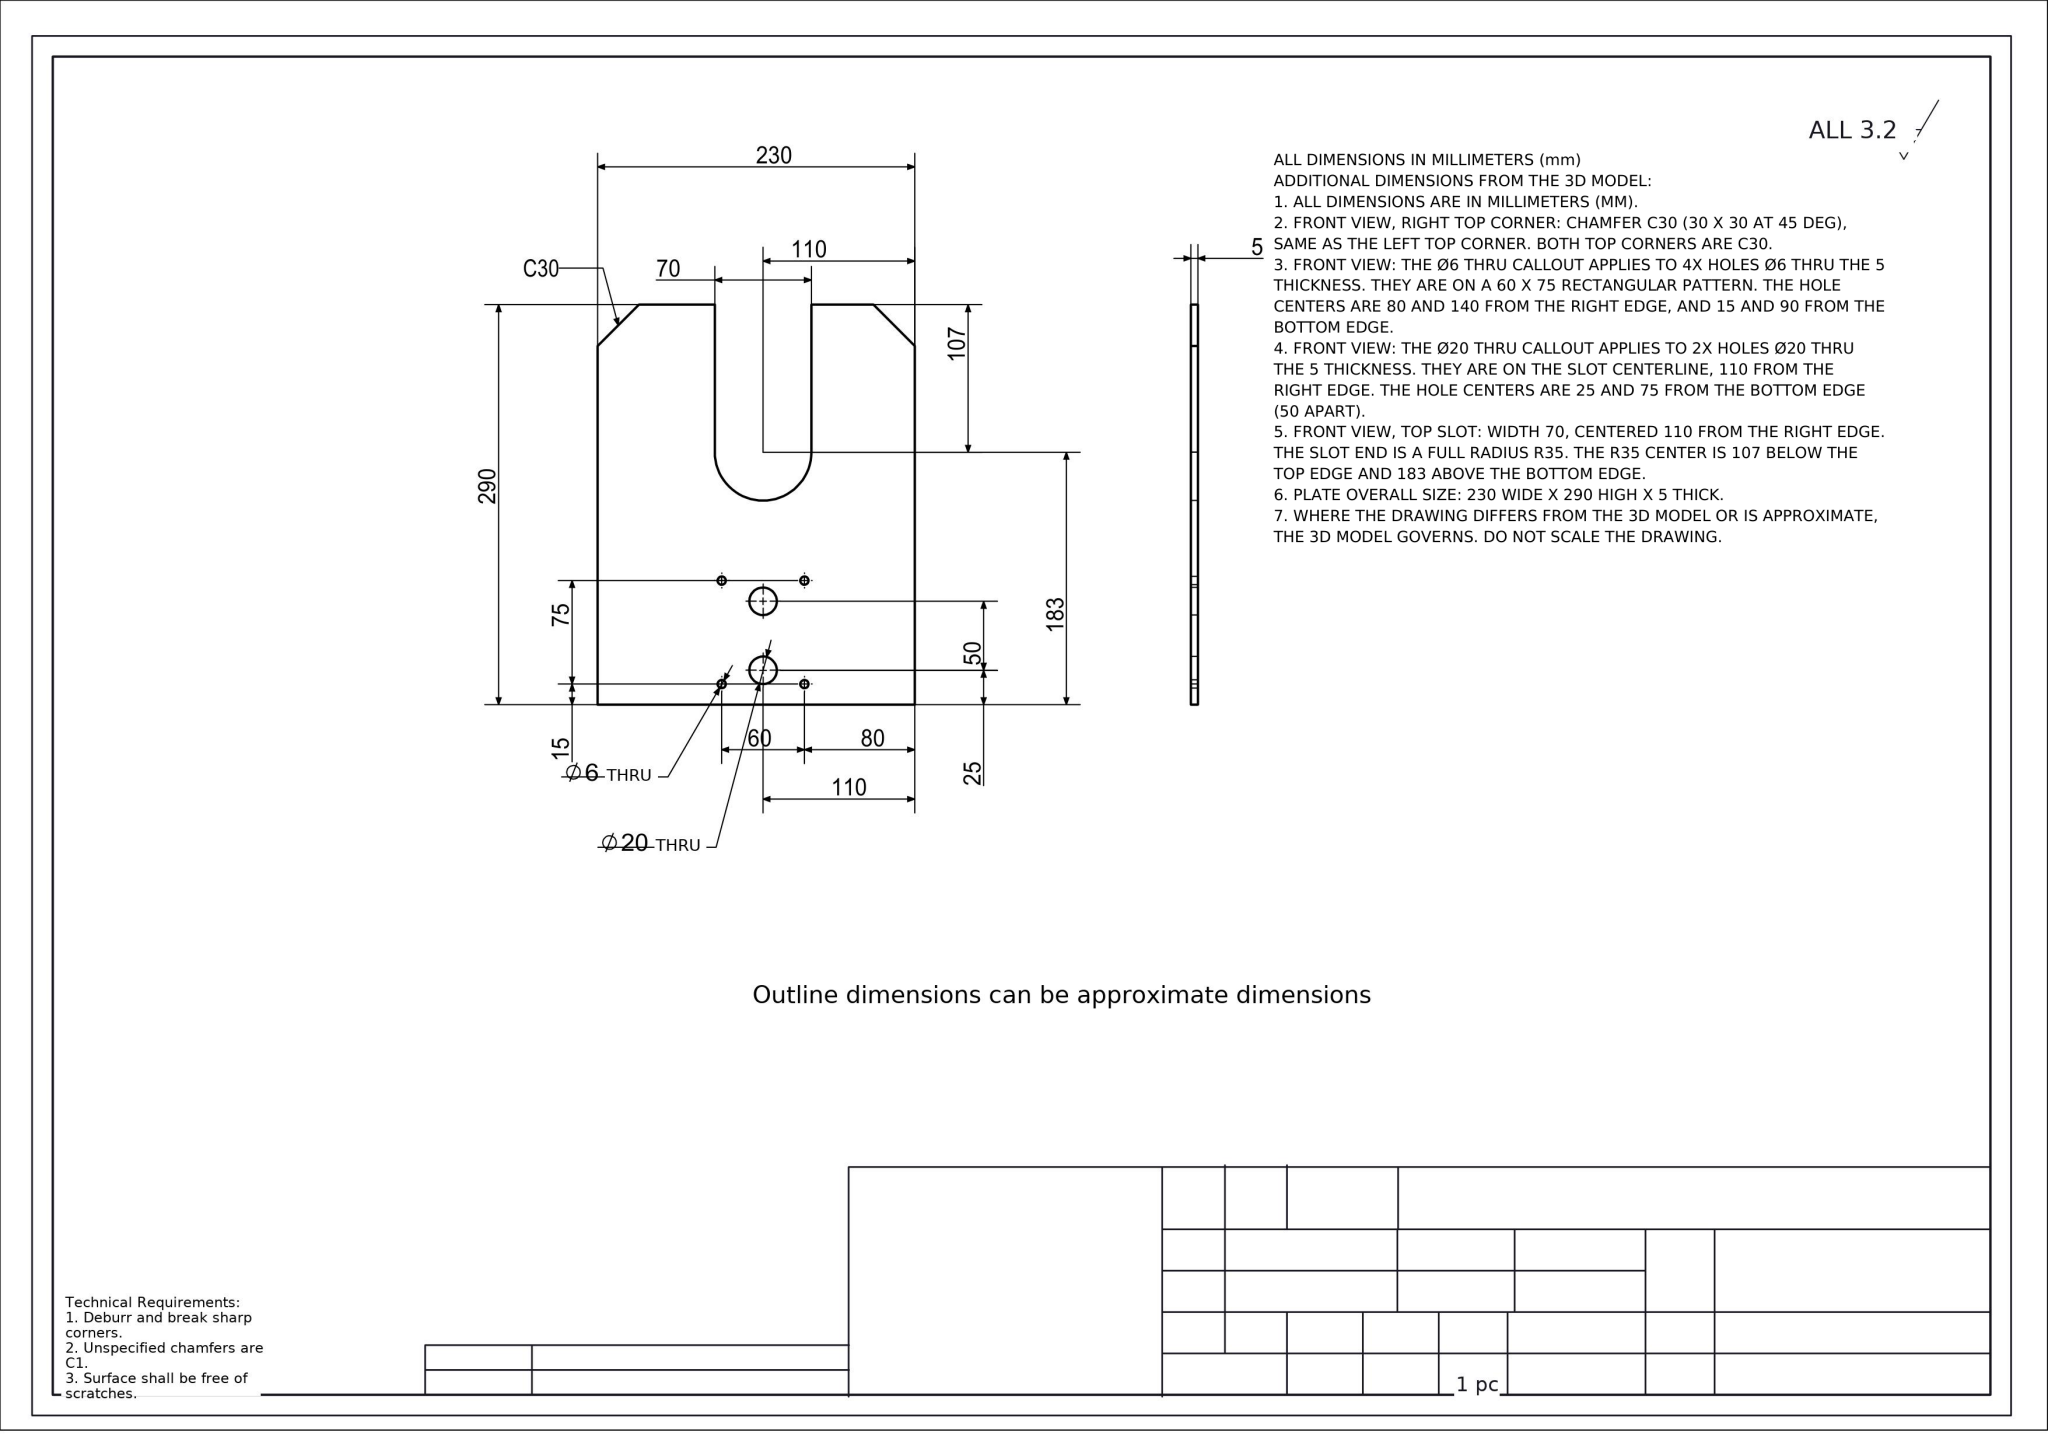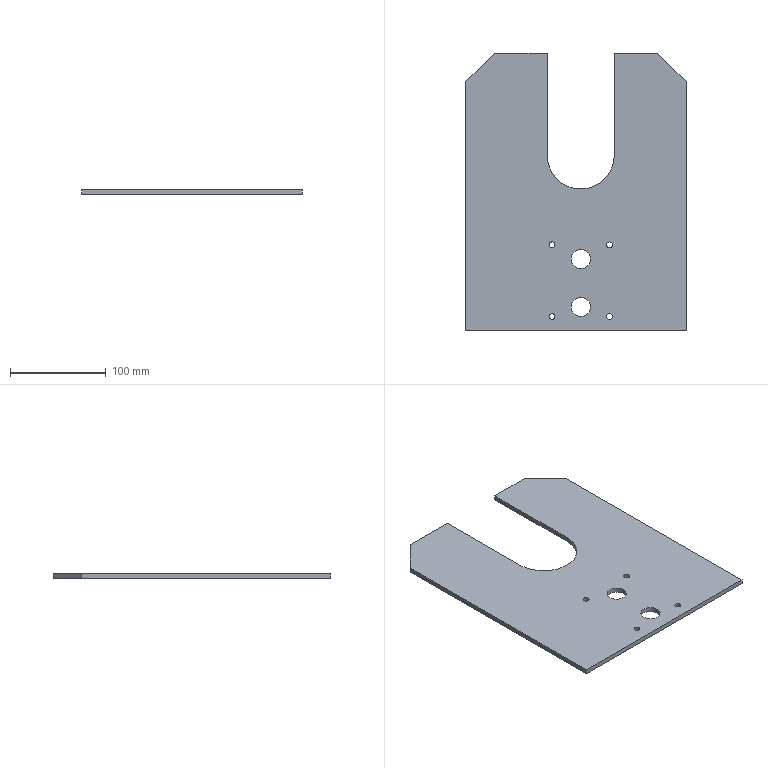Part | NX | mm | U-Notched Multi-Bore Base Plate 230mm | 1 solid | 24 faces | box 230 x 290 x 5 mm | volume 278222 mm3 | cylinder 13 | plane 11 | commonest cylinder face diameters 6 x8 20 x4 70 x1
STEP:
#1=COLOUR_RGB('',0.7922,0.8196,0.9333);
#2=FILL_AREA_STYLE_COLOUR('',#1);
#3=FILL_AREA_STYLE('',(#2));
#4=SURFACE_STYLE_FILL_AREA(#3);
#5=SURFACE_SIDE_STYLE('',(#4));
#6=SURFACE_STYLE_USAGE(.BOTH.,#5);
#7=PRESENTATION_STYLE_ASSIGNMENT((#6));
#8=CARTESIAN_POINT('',(-7.627,5.308,0.));
#9=VERTEX_POINT('',#8);
#10=CARTESIAN_POINT('',(-1.627,5.308,0.));
#11=VERTEX_POINT('',#10);
#12=CARTESIAN_POINT('',(-4.627,5.308,0.));
#13=DIRECTION('',(0.,0.,1.));
#14=DIRECTION('',(1.,0.,0.));
#15=AXIS2_PLACEMENT_3D('',#12,#13,#14);
#16=CIRCLE('',#15,3.);
#17=EDGE_CURVE('',#9,#11,#16,.T.);
#18=ORIENTED_EDGE('',*,*,#17,.F.);
#19=CARTESIAN_POINT('',(-7.627,5.308,5.));
#20=VERTEX_POINT('',#19);
#21=CARTESIAN_POINT('',(-7.627,5.308,0.));
#22=DIRECTION('',(0.,0.,1.));
#23=VECTOR('',#22,1000.);
#24=LINE('',#21,#23);
#25=EDGE_CURVE('',#9,#20,#24,.T.);
#26=ORIENTED_EDGE('',*,*,#25,.T.);
#27=CARTESIAN_POINT('',(-1.627,5.308,5.));
#28=VERTEX_POINT('',#27);
#29=CARTESIAN_POINT('',(-4.627,5.308,5.));
#30=DIRECTION('',(0.,0.,1.));
#31=DIRECTION('',(1.,0.,0.));
#32=AXIS2_PLACEMENT_3D('',#29,#30,#31);
#33=CIRCLE('',#32,3.);
#34=EDGE_CURVE('',#20,#28,#33,.T.);
#35=ORIENTED_EDGE('',*,*,#34,.T.);
#36=CARTESIAN_POINT('',(-1.627,5.308,0.));
#37=DIRECTION('',(0.,0.,1.));
#38=VECTOR('',#37,1000.);
#39=LINE('',#36,#38);
#40=EDGE_CURVE('',#11,#28,#39,.T.);
#41=ORIENTED_EDGE('',*,*,#40,.F.);
#42=EDGE_LOOP('',(#18,#26,#35,#41));
#43=FACE_OUTER_BOUND('',#42,.T.);
#44=CARTESIAN_POINT('',(-4.627,5.308,0.));
#45=DIRECTION('',(0.,0.,1.));
#46=DIRECTION('',(1.,0.,0.));
#47=AXIS2_PLACEMENT_3D('',#44,#45,#46);
#48=CYLINDRICAL_SURFACE('',#47,3.);
#49=ADVANCED_FACE('',(#43),#48,.F.);
#50=CARTESIAN_POINT('',(-7.627,80.308,0.));
#51=VERTEX_POINT('',#50);
#52=CARTESIAN_POINT('',(-1.627,80.308,0.));
#53=VERTEX_POINT('',#52);
#54=CARTESIAN_POINT('',(-4.627,80.308,0.));
#55=DIRECTION('',(0.,0.,1.));
#56=DIRECTION('',(1.,0.,0.));
#57=AXIS2_PLACEMENT_3D('',#54,#55,#56);
#58=CIRCLE('',#57,3.);
#59=EDGE_CURVE('',#51,#53,#58,.T.);
#60=ORIENTED_EDGE('',*,*,#59,.F.);
#61=CARTESIAN_POINT('',(-7.627,80.308,5.));
#62=VERTEX_POINT('',#61);
#63=CARTESIAN_POINT('',(-7.627,80.308,0.));
#64=DIRECTION('',(0.,0.,1.));
#65=VECTOR('',#64,1000.);
#66=LINE('',#63,#65);
#67=EDGE_CURVE('',#51,#62,#66,.T.);
#68=ORIENTED_EDGE('',*,*,#67,.T.);
#69=CARTESIAN_POINT('',(-1.627,80.308,5.));
#70=VERTEX_POINT('',#69);
#71=CARTESIAN_POINT('',(-4.627,80.308,5.));
#72=DIRECTION('',(0.,0.,1.));
#73=DIRECTION('',(1.,0.,0.));
#74=AXIS2_PLACEMENT_3D('',#71,#72,#73);
#75=CIRCLE('',#74,3.);
#76=EDGE_CURVE('',#62,#70,#75,.T.);
#77=ORIENTED_EDGE('',*,*,#76,.T.);
#78=CARTESIAN_POINT('',(-1.627,80.308,0.));
#79=DIRECTION('',(0.,0.,1.));
#80=VECTOR('',#79,1000.);
#81=LINE('',#78,#80);
#82=EDGE_CURVE('',#53,#70,#81,.T.);
#83=ORIENTED_EDGE('',*,*,#82,.F.);
#84=EDGE_LOOP('',(#60,#68,#77,#83));
#85=FACE_OUTER_BOUND('',#84,.T.);
#86=CARTESIAN_POINT('',(-4.627,80.308,0.));
#87=DIRECTION('',(0.,0.,1.));
#88=DIRECTION('',(1.,0.,0.));
#89=AXIS2_PLACEMENT_3D('',#86,#87,#88);
#90=CYLINDRICAL_SURFACE('',#89,3.);
#91=ADVANCED_FACE('',(#85),#90,.F.);
#92=CARTESIAN_POINT('',(52.373,5.308,0.));
#93=VERTEX_POINT('',#92);
#94=CARTESIAN_POINT('',(58.373,5.308,0.));
#95=VERTEX_POINT('',#94);
#96=CARTESIAN_POINT('',(55.373,5.308,0.));
#97=DIRECTION('',(0.,0.,1.));
#98=DIRECTION('',(1.,0.,0.));
#99=AXIS2_PLACEMENT_3D('',#96,#97,#98);
#100=CIRCLE('',#99,3.);
#101=EDGE_CURVE('',#93,#95,#100,.T.);
#102=ORIENTED_EDGE('',*,*,#101,.F.);
#103=CARTESIAN_POINT('',(52.373,5.308,5.));
#104=VERTEX_POINT('',#103);
#105=CARTESIAN_POINT('',(52.373,5.308,0.));
#106=DIRECTION('',(0.,0.,1.));
#107=VECTOR('',#106,1000.);
#108=LINE('',#105,#107);
#109=EDGE_CURVE('',#93,#104,#108,.T.);
#110=ORIENTED_EDGE('',*,*,#109,.T.);
#111=CARTESIAN_POINT('',(58.373,5.308,5.));
#112=VERTEX_POINT('',#111);
#113=CARTESIAN_POINT('',(55.373,5.308,5.));
#114=DIRECTION('',(0.,0.,1.));
#115=DIRECTION('',(1.,0.,0.));
#116=AXIS2_PLACEMENT_3D('',#113,#114,#115);
#117=CIRCLE('',#116,3.);
#118=EDGE_CURVE('',#104,#112,#117,.T.);
#119=ORIENTED_EDGE('',*,*,#118,.T.);
#120=CARTESIAN_POINT('',(58.373,5.308,0.));
#121=DIRECTION('',(0.,0.,1.));
#122=VECTOR('',#121,1000.);
#123=LINE('',#120,#122);
#124=EDGE_CURVE('',#95,#112,#123,.T.);
#125=ORIENTED_EDGE('',*,*,#124,.F.);
#126=EDGE_LOOP('',(#102,#110,#119,#125));
#127=FACE_OUTER_BOUND('',#126,.T.);
#128=CARTESIAN_POINT('',(55.373,5.308,0.));
#129=DIRECTION('',(0.,0.,1.));
#130=DIRECTION('',(1.,0.,0.));
#131=AXIS2_PLACEMENT_3D('',#128,#129,#130);
#132=CYLINDRICAL_SURFACE('',#131,3.);
#133=ADVANCED_FACE('',(#127),#132,.F.);
#134=CARTESIAN_POINT('',(52.373,80.308,0.));
#135=VERTEX_POINT('',#134);
#136=CARTESIAN_POINT('',(58.373,80.308,0.));
#137=VERTEX_POINT('',#136);
#138=CARTESIAN_POINT('',(55.373,80.308,0.));
#139=DIRECTION('',(0.,0.,1.));
#140=DIRECTION('',(1.,0.,0.));
#141=AXIS2_PLACEMENT_3D('',#138,#139,#140);
#142=CIRCLE('',#141,3.);
#143=EDGE_CURVE('',#135,#137,#142,.T.);
#144=ORIENTED_EDGE('',*,*,#143,.F.);
#145=CARTESIAN_POINT('',(52.373,80.308,5.));
#146=VERTEX_POINT('',#145);
#147=CARTESIAN_POINT('',(52.373,80.308,0.));
#148=DIRECTION('',(0.,0.,1.));
#149=VECTOR('',#148,1000.);
#150=LINE('',#147,#149);
#151=EDGE_CURVE('',#135,#146,#150,.T.);
#152=ORIENTED_EDGE('',*,*,#151,.T.);
#153=CARTESIAN_POINT('',(58.373,80.308,5.));
#154=VERTEX_POINT('',#153);
#155=CARTESIAN_POINT('',(55.373,80.308,5.));
#156=DIRECTION('',(0.,0.,1.));
#157=DIRECTION('',(1.,0.,0.));
#158=AXIS2_PLACEMENT_3D('',#155,#156,#157);
#159=CIRCLE('',#158,3.);
#160=EDGE_CURVE('',#146,#154,#159,.T.);
#161=ORIENTED_EDGE('',*,*,#160,.T.);
#162=CARTESIAN_POINT('',(58.373,80.308,0.));
#163=DIRECTION('',(0.,0.,1.));
#164=VECTOR('',#163,1000.);
#165=LINE('',#162,#164);
#166=EDGE_CURVE('',#137,#154,#165,.T.);
#167=ORIENTED_EDGE('',*,*,#166,.F.);
#168=EDGE_LOOP('',(#144,#152,#161,#167));
#169=FACE_OUTER_BOUND('',#168,.T.);
#170=CARTESIAN_POINT('',(55.373,80.308,0.));
#171=DIRECTION('',(0.,0.,1.));
#172=DIRECTION('',(1.,0.,0.));
#173=AXIS2_PLACEMENT_3D('',#170,#171,#172);
#174=CYLINDRICAL_SURFACE('',#173,3.);
#175=ADVANCED_FACE('',(#169),#174,.F.);
#176=CARTESIAN_POINT('',(15.373,65.308,0.));
#177=VERTEX_POINT('',#176);
#178=CARTESIAN_POINT('',(35.373,65.308,0.));
#179=VERTEX_POINT('',#178);
#180=CARTESIAN_POINT('',(25.373,65.308,0.));
#181=DIRECTION('',(0.,0.,1.));
#182=DIRECTION('',(1.,0.,0.));
#183=AXIS2_PLACEMENT_3D('',#180,#181,#182);
#184=CIRCLE('',#183,10.);
#185=EDGE_CURVE('',#177,#179,#184,.T.);
#186=ORIENTED_EDGE('',*,*,#185,.F.);
#187=CARTESIAN_POINT('',(15.373,65.308,5.));
#188=VERTEX_POINT('',#187);
#189=CARTESIAN_POINT('',(15.373,65.308,0.));
#190=DIRECTION('',(0.,0.,1.));
#191=VECTOR('',#190,1000.);
#192=LINE('',#189,#191);
#193=EDGE_CURVE('',#177,#188,#192,.T.);
#194=ORIENTED_EDGE('',*,*,#193,.T.);
#195=CARTESIAN_POINT('',(35.373,65.308,5.));
#196=VERTEX_POINT('',#195);
#197=CARTESIAN_POINT('',(25.373,65.308,5.));
#198=DIRECTION('',(0.,0.,1.));
#199=DIRECTION('',(1.,0.,0.));
#200=AXIS2_PLACEMENT_3D('',#197,#198,#199);
#201=CIRCLE('',#200,10.);
#202=EDGE_CURVE('',#188,#196,#201,.T.);
#203=ORIENTED_EDGE('',*,*,#202,.T.);
#204=CARTESIAN_POINT('',(35.373,65.308,0.));
#205=DIRECTION('',(0.,0.,1.));
#206=VECTOR('',#205,1000.);
#207=LINE('',#204,#206);
#208=EDGE_CURVE('',#179,#196,#207,.T.);
#209=ORIENTED_EDGE('',*,*,#208,.F.);
#210=EDGE_LOOP('',(#186,#194,#203,#209));
#211=FACE_OUTER_BOUND('',#210,.T.);
#212=CARTESIAN_POINT('',(25.373,65.308,0.));
#213=DIRECTION('',(0.,0.,1.));
#214=DIRECTION('',(1.,0.,0.));
#215=AXIS2_PLACEMENT_3D('',#212,#213,#214);
#216=CYLINDRICAL_SURFACE('',#215,10.);
#217=ADVANCED_FACE('',(#211),#216,.F.);
#218=CARTESIAN_POINT('',(15.373,15.308,0.));
#219=VERTEX_POINT('',#218);
#220=CARTESIAN_POINT('',(35.373,15.308,0.));
#221=VERTEX_POINT('',#220);
#222=CARTESIAN_POINT('',(25.373,15.308,0.));
#223=DIRECTION('',(0.,0.,1.));
#224=DIRECTION('',(1.,0.,0.));
#225=AXIS2_PLACEMENT_3D('',#222,#223,#224);
#226=CIRCLE('',#225,10.);
#227=EDGE_CURVE('',#219,#221,#226,.T.);
#228=ORIENTED_EDGE('',*,*,#227,.F.);
#229=CARTESIAN_POINT('',(15.373,15.308,5.));
#230=VERTEX_POINT('',#229);
#231=CARTESIAN_POINT('',(15.373,15.308,0.));
#232=DIRECTION('',(0.,0.,1.));
#233=VECTOR('',#232,1000.);
#234=LINE('',#231,#233);
#235=EDGE_CURVE('',#219,#230,#234,.T.);
#236=ORIENTED_EDGE('',*,*,#235,.T.);
#237=CARTESIAN_POINT('',(35.373,15.308,5.));
#238=VERTEX_POINT('',#237);
#239=CARTESIAN_POINT('',(25.373,15.308,5.));
#240=DIRECTION('',(0.,0.,1.));
#241=DIRECTION('',(1.,0.,0.));
#242=AXIS2_PLACEMENT_3D('',#239,#240,#241);
#243=CIRCLE('',#242,10.);
#244=EDGE_CURVE('',#230,#238,#243,.T.);
#245=ORIENTED_EDGE('',*,*,#244,.T.);
#246=CARTESIAN_POINT('',(35.373,15.308,0.));
#247=DIRECTION('',(0.,0.,1.));
#248=VECTOR('',#247,1000.);
#249=LINE('',#246,#248);
#250=EDGE_CURVE('',#221,#238,#249,.T.);
#251=ORIENTED_EDGE('',*,*,#250,.F.);
#252=EDGE_LOOP('',(#228,#236,#245,#251));
#253=FACE_OUTER_BOUND('',#252,.T.);
#254=CARTESIAN_POINT('',(25.373,15.308,0.));
#255=DIRECTION('',(0.,0.,1.));
#256=DIRECTION('',(1.,0.,0.));
#257=AXIS2_PLACEMENT_3D('',#254,#255,#256);
#258=CYLINDRICAL_SURFACE('',#257,10.);
#259=ADVANCED_FACE('',(#253),#258,.F.);
#260=CARTESIAN_POINT('',(-9.627,280.308,0.));
#261=VERTEX_POINT('',#260);
#262=CARTESIAN_POINT('',(-64.627,280.308,0.));
#263=VERTEX_POINT('',#262);
#264=CARTESIAN_POINT('',(-94.627,280.308,0.));
#265=DIRECTION('',(-1.,0.,0.));
#266=VECTOR('',#265,1000.);
#267=LINE('',#264,#266);
#268=EDGE_CURVE('',#261,#263,#267,.T.);
#269=ORIENTED_EDGE('',*,*,#268,.T.);
#270=CARTESIAN_POINT('',(-64.627,280.308,5.));
#271=VERTEX_POINT('',#270);
#272=CARTESIAN_POINT('',(-64.627,280.308,5.));
#273=DIRECTION('',(0.,0.,1.));
#274=VECTOR('',#273,1000.);
#275=LINE('',#272,#274);
#276=EDGE_CURVE('',#263,#271,#275,.T.);
#277=ORIENTED_EDGE('',*,*,#276,.T.);
#278=CARTESIAN_POINT('',(-9.627,280.308,5.));
#279=VERTEX_POINT('',#278);
#280=CARTESIAN_POINT('',(-94.627,280.308,5.));
#281=DIRECTION('',(-1.,0.,0.));
#282=VECTOR('',#281,1000.);
#283=LINE('',#280,#282);
#284=EDGE_CURVE('',#279,#271,#283,.T.);
#285=ORIENTED_EDGE('',*,*,#284,.F.);
#286=CARTESIAN_POINT('',(-9.627,280.308,0.));
#287=DIRECTION('',(0.,0.,1.));
#288=VECTOR('',#287,1000.);
#289=LINE('',#286,#288);
#290=EDGE_CURVE('',#261,#279,#289,.T.);
#291=ORIENTED_EDGE('',*,*,#290,.F.);
#292=EDGE_LOOP('',(#269,#277,#285,#291));
#293=FACE_OUTER_BOUND('',#292,.T.);
#294=CARTESIAN_POINT('',(-94.627,280.308,5.));
#295=DIRECTION('',(0.,-1.,0.));
#296=DIRECTION('',(0.,0.,-1.));
#297=AXIS2_PLACEMENT_3D('',#294,#295,#296);
#298=PLANE('',#297);
#299=ADVANCED_FACE('',(#293),#298,.F.);
#300=CARTESIAN_POINT('',(-94.627,250.308,5.));
#301=VERTEX_POINT('',#300);
#302=CARTESIAN_POINT('',(-94.627,-9.692,5.));
#303=VERTEX_POINT('',#302);
#304=CARTESIAN_POINT('',(-94.627,-9.692,5.));
#305=DIRECTION('',(0.,-1.,0.));
#306=VECTOR('',#305,1000.);
#307=LINE('',#304,#306);
#308=EDGE_CURVE('',#301,#303,#307,.T.);
#309=ORIENTED_EDGE('',*,*,#308,.F.);
#310=CARTESIAN_POINT('',(-94.627,250.308,0.));
#311=VERTEX_POINT('',#310);
#312=CARTESIAN_POINT('',(-94.627,250.308,5.));
#313=DIRECTION('',(0.,0.,-1.));
#314=VECTOR('',#313,1000.);
#315=LINE('',#312,#314);
#316=EDGE_CURVE('',#301,#311,#315,.T.);
#317=ORIENTED_EDGE('',*,*,#316,.T.);
#318=CARTESIAN_POINT('',(-94.627,-9.692,0.));
#319=VERTEX_POINT('',#318);
#320=CARTESIAN_POINT('',(-94.627,-9.692,0.));
#321=DIRECTION('',(0.,-1.,0.));
#322=VECTOR('',#321,1000.);
#323=LINE('',#320,#322);
#324=EDGE_CURVE('',#311,#319,#323,.T.);
#325=ORIENTED_EDGE('',*,*,#324,.T.);
#326=CARTESIAN_POINT('',(-94.627,-9.692,5.));
#327=DIRECTION('',(0.,0.,-1.));
#328=VECTOR('',#327,1000.);
#329=LINE('',#326,#328);
#330=EDGE_CURVE('',#303,#319,#329,.T.);
#331=ORIENTED_EDGE('',*,*,#330,.F.);
#332=EDGE_LOOP('',(#309,#317,#325,#331));
#333=FACE_OUTER_BOUND('',#332,.T.);
#334=CARTESIAN_POINT('',(-94.627,-9.692,5.));
#335=DIRECTION('',(1.,0.,0.));
#336=DIRECTION('',(0.,0.,-1.));
#337=AXIS2_PLACEMENT_3D('',#334,#335,#336);
#338=PLANE('',#337);
#339=ADVANCED_FACE('',(#333),#338,.F.);
#340=CARTESIAN_POINT('',(135.373,-9.692,0.));
#341=VERTEX_POINT('',#340);
#342=CARTESIAN_POINT('',(-94.627,-9.692,0.));
#343=DIRECTION('',(1.,0.,0.));
#344=VECTOR('',#343,1000.);
#345=LINE('',#342,#344);
#346=EDGE_CURVE('',#319,#341,#345,.T.);
#347=ORIENTED_EDGE('',*,*,#346,.T.);
#348=CARTESIAN_POINT('',(135.373,-9.692,5.));
#349=VERTEX_POINT('',#348);
#350=CARTESIAN_POINT('',(135.373,-9.692,5.));
#351=DIRECTION('',(0.,0.,-1.));
#352=VECTOR('',#351,1000.);
#353=LINE('',#350,#352);
#354=EDGE_CURVE('',#349,#341,#353,.T.);
#355=ORIENTED_EDGE('',*,*,#354,.F.);
#356=CARTESIAN_POINT('',(-94.627,-9.692,5.));
#357=DIRECTION('',(1.,0.,0.));
#358=VECTOR('',#357,1000.);
#359=LINE('',#356,#358);
#360=EDGE_CURVE('',#303,#349,#359,.T.);
#361=ORIENTED_EDGE('',*,*,#360,.F.);
#362=ORIENTED_EDGE('',*,*,#330,.T.);
#363=EDGE_LOOP('',(#347,#355,#361,#362));
#364=FACE_OUTER_BOUND('',#363,.T.);
#365=CARTESIAN_POINT('',(-94.627,-9.692,5.));
#366=DIRECTION('',(0.,1.,0.));
#367=DIRECTION('',(0.,0.,1.));
#368=AXIS2_PLACEMENT_3D('',#365,#366,#367);
#369=PLANE('',#368);
#370=ADVANCED_FACE('',(#364),#369,.F.);
#371=CARTESIAN_POINT('',(135.373,250.308,0.));
#372=VERTEX_POINT('',#371);
#373=CARTESIAN_POINT('',(135.373,-9.692,0.));
#374=DIRECTION('',(0.,1.,0.));
#375=VECTOR('',#374,1000.);
#376=LINE('',#373,#375);
#377=EDGE_CURVE('',#341,#372,#376,.T.);
#378=ORIENTED_EDGE('',*,*,#377,.T.);
#379=CARTESIAN_POINT('',(135.373,250.308,5.));
#380=VERTEX_POINT('',#379);
#381=CARTESIAN_POINT('',(135.373,250.308,5.));
#382=DIRECTION('',(0.,0.,1.));
#383=VECTOR('',#382,1000.);
#384=LINE('',#381,#383);
#385=EDGE_CURVE('',#372,#380,#384,.T.);
#386=ORIENTED_EDGE('',*,*,#385,.T.);
#387=CARTESIAN_POINT('',(135.373,-9.692,5.));
#388=DIRECTION('',(0.,1.,0.));
#389=VECTOR('',#388,1000.);
#390=LINE('',#387,#389);
#391=EDGE_CURVE('',#349,#380,#390,.T.);
#392=ORIENTED_EDGE('',*,*,#391,.F.);
#393=ORIENTED_EDGE('',*,*,#354,.T.);
#394=EDGE_LOOP('',(#378,#386,#392,#393));
#395=FACE_OUTER_BOUND('',#394,.T.);
#396=CARTESIAN_POINT('',(135.373,-9.692,5.));
#397=DIRECTION('',(-1.,0.,0.));
#398=DIRECTION('',(0.,0.,1.));
#399=AXIS2_PLACEMENT_3D('',#396,#397,#398);
#400=PLANE('',#399);
#401=ADVANCED_FACE('',(#395),#400,.F.);
#402=CARTESIAN_POINT('',(105.373,280.308,5.));
#403=VERTEX_POINT('',#402);
#404=CARTESIAN_POINT('',(60.373,280.308,5.));
#405=VERTEX_POINT('',#404);
#406=CARTESIAN_POINT('',(-94.627,280.308,5.));
#407=DIRECTION('',(-1.,0.,0.));
#408=VECTOR('',#407,1000.);
#409=LINE('',#406,#408);
#410=EDGE_CURVE('',#403,#405,#409,.T.);
#411=ORIENTED_EDGE('',*,*,#410,.F.);
#412=CARTESIAN_POINT('',(105.373,280.308,0.));
#413=VERTEX_POINT('',#412);
#414=CARTESIAN_POINT('',(105.373,280.308,5.));
#415=DIRECTION('',(0.,0.,-1.));
#416=VECTOR('',#415,1000.);
#417=LINE('',#414,#416);
#418=EDGE_CURVE('',#403,#413,#417,.T.);
#419=ORIENTED_EDGE('',*,*,#418,.T.);
#420=CARTESIAN_POINT('',(60.373,280.308,0.));
#421=VERTEX_POINT('',#420);
#422=CARTESIAN_POINT('',(-94.627,280.308,0.));
#423=DIRECTION('',(-1.,0.,0.));
#424=VECTOR('',#423,1000.);
#425=LINE('',#422,#424);
#426=EDGE_CURVE('',#413,#421,#425,.T.);
#427=ORIENTED_EDGE('',*,*,#426,.T.);
#428=CARTESIAN_POINT('',(60.373,280.308,0.));
#429=DIRECTION('',(0.,0.,1.));
#430=VECTOR('',#429,1000.);
#431=LINE('',#428,#430);
#432=EDGE_CURVE('',#421,#405,#431,.T.);
#433=ORIENTED_EDGE('',*,*,#432,.T.);
#434=EDGE_LOOP('',(#411,#419,#427,#433));
#435=FACE_OUTER_BOUND('',#434,.T.);
#436=CARTESIAN_POINT('',(-94.627,280.308,5.));
#437=DIRECTION('',(0.,-1.,0.));
#438=DIRECTION('',(0.,0.,-1.));
#439=AXIS2_PLACEMENT_3D('',#436,#437,#438);
#440=PLANE('',#439);
#441=ADVANCED_FACE('',(#435),#440,.F.);
#442=CARTESIAN_POINT('',(-4.627,5.308,5.));
#443=DIRECTION('',(0.,0.,1.));
#444=DIRECTION('',(1.,0.,0.));
#445=AXIS2_PLACEMENT_3D('',#442,#443,#444);
#446=CIRCLE('',#445,3.);
#447=EDGE_CURVE('',#28,#20,#446,.T.);
#448=ORIENTED_EDGE('',*,*,#447,.F.);
#449=ORIENTED_EDGE('',*,*,#34,.F.);
#450=EDGE_LOOP('',(#448,#449));
#451=FACE_BOUND('',#450,.T.);
#452=CARTESIAN_POINT('',(-4.627,80.308,5.));
#453=DIRECTION('',(0.,0.,1.));
#454=DIRECTION('',(1.,0.,0.));
#455=AXIS2_PLACEMENT_3D('',#452,#453,#454);
#456=CIRCLE('',#455,3.);
#457=EDGE_CURVE('',#70,#62,#456,.T.);
#458=ORIENTED_EDGE('',*,*,#457,.F.);
#459=ORIENTED_EDGE('',*,*,#76,.F.);
#460=EDGE_LOOP('',(#458,#459));
#461=FACE_BOUND('',#460,.T.);
#462=CARTESIAN_POINT('',(55.373,5.308,5.));
#463=DIRECTION('',(0.,0.,1.));
#464=DIRECTION('',(1.,0.,0.));
#465=AXIS2_PLACEMENT_3D('',#462,#463,#464);
#466=CIRCLE('',#465,3.);
#467=EDGE_CURVE('',#112,#104,#466,.T.);
#468=ORIENTED_EDGE('',*,*,#467,.F.);
#469=ORIENTED_EDGE('',*,*,#118,.F.);
#470=EDGE_LOOP('',(#468,#469));
#471=FACE_BOUND('',#470,.T.);
#472=CARTESIAN_POINT('',(55.373,80.308,5.));
#473=DIRECTION('',(0.,0.,1.));
#474=DIRECTION('',(1.,0.,0.));
#475=AXIS2_PLACEMENT_3D('',#472,#473,#474);
#476=CIRCLE('',#475,3.);
#477=EDGE_CURVE('',#154,#146,#476,.T.);
#478=ORIENTED_EDGE('',*,*,#477,.F.);
#479=ORIENTED_EDGE('',*,*,#160,.F.);
#480=EDGE_LOOP('',(#478,#479));
#481=FACE_BOUND('',#480,.T.);
#482=CARTESIAN_POINT('',(25.373,65.308,5.));
#483=DIRECTION('',(0.,0.,1.));
#484=DIRECTION('',(1.,0.,0.));
#485=AXIS2_PLACEMENT_3D('',#482,#483,#484);
#486=CIRCLE('',#485,10.);
#487=EDGE_CURVE('',#196,#188,#486,.T.);
#488=ORIENTED_EDGE('',*,*,#487,.F.);
#489=ORIENTED_EDGE('',*,*,#202,.F.);
#490=EDGE_LOOP('',(#488,#489));
#491=FACE_BOUND('',#490,.T.);
#492=CARTESIAN_POINT('',(25.373,15.308,5.));
#493=DIRECTION('',(0.,0.,1.));
#494=DIRECTION('',(1.,0.,0.));
#495=AXIS2_PLACEMENT_3D('',#492,#493,#494);
#496=CIRCLE('',#495,10.);
#497=EDGE_CURVE('',#238,#230,#496,.T.);
#498=ORIENTED_EDGE('',*,*,#497,.F.);
#499=ORIENTED_EDGE('',*,*,#244,.F.);
#500=EDGE_LOOP('',(#498,#499));
#501=FACE_BOUND('',#500,.T.);
#502=ORIENTED_EDGE('',*,*,#391,.T.);
#503=CARTESIAN_POINT('',(105.373,280.308,5.));
#504=DIRECTION('',(-0.7071,0.7071,0.));
#505=VECTOR('',#504,1000.);
#506=LINE('',#503,#505);
#507=EDGE_CURVE('',#380,#403,#506,.T.);
#508=ORIENTED_EDGE('',*,*,#507,.T.);
#509=ORIENTED_EDGE('',*,*,#410,.T.);
#510=CARTESIAN_POINT('',(60.373,173.308,5.));
#511=VERTEX_POINT('',#510);
#512=CARTESIAN_POINT('',(60.373,173.308,5.));
#513=DIRECTION('',(0.,1.,0.));
#514=VECTOR('',#513,1000.);
#515=LINE('',#512,#514);
#516=EDGE_CURVE('',#511,#405,#515,.T.);
#517=ORIENTED_EDGE('',*,*,#516,.F.);
#518=CARTESIAN_POINT('',(-9.627,173.308,5.));
#519=VERTEX_POINT('',#518);
#520=CARTESIAN_POINT('',(25.373,173.308,5.));
#521=DIRECTION('',(0.,0.,1.));
#522=DIRECTION('',(1.,0.,0.));
#523=AXIS2_PLACEMENT_3D('',#520,#521,#522);
#524=CIRCLE('',#523,35.);
#525=EDGE_CURVE('',#519,#511,#524,.T.);
#526=ORIENTED_EDGE('',*,*,#525,.F.);
#527=CARTESIAN_POINT('',(-9.627,173.308,5.));
#528=DIRECTION('',(0.,-1.,0.));
#529=VECTOR('',#528,1000.);
#530=LINE('',#527,#529);
#531=EDGE_CURVE('',#279,#519,#530,.T.);
#532=ORIENTED_EDGE('',*,*,#531,.F.);
#533=ORIENTED_EDGE('',*,*,#284,.T.);
#534=CARTESIAN_POINT('',(-94.627,250.308,5.));
#535=DIRECTION('',(-0.7071,-0.7071,0.));
#536=VECTOR('',#535,1000.);
#537=LINE('',#534,#536);
#538=EDGE_CURVE('',#271,#301,#537,.T.);
#539=ORIENTED_EDGE('',*,*,#538,.T.);
#540=ORIENTED_EDGE('',*,*,#308,.T.);
#541=ORIENTED_EDGE('',*,*,#360,.T.);
#542=EDGE_LOOP('',(#502,#508,#509,#517,#526,#532,#533,#539,#540,#541));
#543=FACE_OUTER_BOUND('',#542,.T.);
#544=CARTESIAN_POINT('',(0.,0.,5.));
#545=DIRECTION('',(0.,0.,-1.));
#546=DIRECTION('',(-1.,0.,0.));
#547=AXIS2_PLACEMENT_3D('',#544,#545,#546);
#548=PLANE('',#547);
#549=ADVANCED_FACE('',(#451,#461,#471,#481,#491,#501,#543),#548,.F.);
#550=CARTESIAN_POINT('',(-4.627,5.308,0.));
#551=DIRECTION('',(0.,0.,1.));
#552=DIRECTION('',(1.,0.,0.));
#553=AXIS2_PLACEMENT_3D('',#550,#551,#552);
#554=CIRCLE('',#553,3.);
#555=EDGE_CURVE('',#11,#9,#554,.T.);
#556=ORIENTED_EDGE('',*,*,#555,.T.);
#557=ORIENTED_EDGE('',*,*,#17,.T.);
#558=EDGE_LOOP('',(#556,#557));
#559=FACE_BOUND('',#558,.T.);
#560=CARTESIAN_POINT('',(-4.627,80.308,0.));
#561=DIRECTION('',(0.,0.,1.));
#562=DIRECTION('',(1.,0.,0.));
#563=AXIS2_PLACEMENT_3D('',#560,#561,#562);
#564=CIRCLE('',#563,3.);
#565=EDGE_CURVE('',#53,#51,#564,.T.);
#566=ORIENTED_EDGE('',*,*,#565,.T.);
#567=ORIENTED_EDGE('',*,*,#59,.T.);
#568=EDGE_LOOP('',(#566,#567));
#569=FACE_BOUND('',#568,.T.);
#570=CARTESIAN_POINT('',(55.373,5.308,0.));
#571=DIRECTION('',(0.,0.,1.));
#572=DIRECTION('',(1.,0.,0.));
#573=AXIS2_PLACEMENT_3D('',#570,#571,#572);
#574=CIRCLE('',#573,3.);
#575=EDGE_CURVE('',#95,#93,#574,.T.);
#576=ORIENTED_EDGE('',*,*,#575,.T.);
#577=ORIENTED_EDGE('',*,*,#101,.T.);
#578=EDGE_LOOP('',(#576,#577));
#579=FACE_BOUND('',#578,.T.);
#580=CARTESIAN_POINT('',(55.373,80.308,0.));
#581=DIRECTION('',(0.,0.,1.));
#582=DIRECTION('',(1.,0.,0.));
#583=AXIS2_PLACEMENT_3D('',#580,#581,#582);
#584=CIRCLE('',#583,3.);
#585=EDGE_CURVE('',#137,#135,#584,.T.);
#586=ORIENTED_EDGE('',*,*,#585,.T.);
#587=ORIENTED_EDGE('',*,*,#143,.T.);
#588=EDGE_LOOP('',(#586,#587));
#589=FACE_BOUND('',#588,.T.);
#590=ORIENTED_EDGE('',*,*,#426,.F.);
#591=CARTESIAN_POINT('',(192.841,192.841,0.));
#592=DIRECTION('',(0.7071,-0.7071,0.));
#593=VECTOR('',#592,1000.);
#594=LINE('',#591,#593);
#595=EDGE_CURVE('',#413,#372,#594,.T.);
#596=ORIENTED_EDGE('',*,*,#595,.T.);
#597=ORIENTED_EDGE('',*,*,#377,.F.);
#598=ORIENTED_EDGE('',*,*,#346,.F.);
#599=ORIENTED_EDGE('',*,*,#324,.F.);
#600=CARTESIAN_POINT('',(-172.468,172.468,0.));
#601=DIRECTION('',(0.7071,0.7071,0.));
#602=VECTOR('',#601,1000.);
#603=LINE('',#600,#602);
#604=EDGE_CURVE('',#311,#263,#603,.T.);
#605=ORIENTED_EDGE('',*,*,#604,.T.);
#606=ORIENTED_EDGE('',*,*,#268,.F.);
#607=CARTESIAN_POINT('',(-9.627,173.308,0.));
#608=VERTEX_POINT('',#607);
#609=CARTESIAN_POINT('',(-9.627,173.308,0.));
#610=DIRECTION('',(0.,-1.,0.));
#611=VECTOR('',#610,1000.);
#612=LINE('',#609,#611);
#613=EDGE_CURVE('',#261,#608,#612,.T.);
#614=ORIENTED_EDGE('',*,*,#613,.T.);
#615=CARTESIAN_POINT('',(60.373,173.308,0.));
#616=VERTEX_POINT('',#615);
#617=CARTESIAN_POINT('',(25.373,173.308,0.));
#618=DIRECTION('',(0.,0.,1.));
#619=DIRECTION('',(1.,0.,0.));
#620=AXIS2_PLACEMENT_3D('',#617,#618,#619);
#621=CIRCLE('',#620,35.);
#622=EDGE_CURVE('',#608,#616,#621,.T.);
#623=ORIENTED_EDGE('',*,*,#622,.T.);
#624=CARTESIAN_POINT('',(60.373,173.308,0.));
#625=DIRECTION('',(0.,1.,0.));
#626=VECTOR('',#625,1000.);
#627=LINE('',#624,#626);
#628=EDGE_CURVE('',#616,#421,#627,.T.);
#629=ORIENTED_EDGE('',*,*,#628,.T.);
#630=EDGE_LOOP('',(#590,#596,#597,#598,#599,#605,#606,#614,#623,#629));
#631=FACE_OUTER_BOUND('',#630,.T.);
#632=CARTESIAN_POINT('',(25.373,65.308,0.));
#633=DIRECTION('',(0.,0.,1.));
#634=DIRECTION('',(1.,0.,0.));
#635=AXIS2_PLACEMENT_3D('',#632,#633,#634);
#636=CIRCLE('',#635,10.);
#637=EDGE_CURVE('',#179,#177,#636,.T.);
#638=ORIENTED_EDGE('',*,*,#637,.T.);
#639=ORIENTED_EDGE('',*,*,#185,.T.);
#640=EDGE_LOOP('',(#638,#639));
#641=FACE_BOUND('',#640,.T.);
#642=CARTESIAN_POINT('',(25.373,15.308,0.));
#643=DIRECTION('',(0.,0.,1.));
#644=DIRECTION('',(1.,0.,0.));
#645=AXIS2_PLACEMENT_3D('',#642,#643,#644);
#646=CIRCLE('',#645,10.);
#647=EDGE_CURVE('',#221,#219,#646,.T.);
#648=ORIENTED_EDGE('',*,*,#647,.T.);
#649=ORIENTED_EDGE('',*,*,#227,.T.);
#650=EDGE_LOOP('',(#648,#649));
#651=FACE_BOUND('',#650,.T.);
#652=CARTESIAN_POINT('',(0.,0.,0.));
#653=DIRECTION('',(0.,0.,-1.));
#654=DIRECTION('',(-1.,0.,0.));
#655=AXIS2_PLACEMENT_3D('',#652,#653,#654);
#656=PLANE('',#655);
#657=ADVANCED_FACE('',(#559,#569,#579,#589,#631,#641,#651),#656,.T.);
#658=ORIENTED_EDGE('',*,*,#235,.F.);
#659=ORIENTED_EDGE('',*,*,#647,.F.);
#660=ORIENTED_EDGE('',*,*,#250,.T.);
#661=ORIENTED_EDGE('',*,*,#497,.T.);
#662=EDGE_LOOP('',(#658,#659,#660,#661));
#663=FACE_OUTER_BOUND('',#662,.T.);
#664=CARTESIAN_POINT('',(25.373,15.308,0.));
#665=DIRECTION('',(0.,0.,1.));
#666=DIRECTION('',(1.,0.,0.));
#667=AXIS2_PLACEMENT_3D('',#664,#665,#666);
#668=CYLINDRICAL_SURFACE('',#667,10.);
#669=ADVANCED_FACE('',(#663),#668,.F.);
#670=ORIENTED_EDGE('',*,*,#193,.F.);
#671=ORIENTED_EDGE('',*,*,#637,.F.);
#672=ORIENTED_EDGE('',*,*,#208,.T.);
#673=ORIENTED_EDGE('',*,*,#487,.T.);
#674=EDGE_LOOP('',(#670,#671,#672,#673));
#675=FACE_OUTER_BOUND('',#674,.T.);
#676=CARTESIAN_POINT('',(25.373,65.308,0.));
#677=DIRECTION('',(0.,0.,1.));
#678=DIRECTION('',(1.,0.,0.));
#679=AXIS2_PLACEMENT_3D('',#676,#677,#678);
#680=CYLINDRICAL_SURFACE('',#679,10.);
#681=ADVANCED_FACE('',(#675),#680,.F.);
#682=ORIENTED_EDGE('',*,*,#525,.T.);
#683=CARTESIAN_POINT('',(60.373,173.308,0.));
#684=DIRECTION('',(0.,0.,1.));
#685=VECTOR('',#684,1000.);
#686=LINE('',#683,#685);
#687=EDGE_CURVE('',#616,#511,#686,.T.);
#688=ORIENTED_EDGE('',*,*,#687,.F.);
#689=ORIENTED_EDGE('',*,*,#622,.F.);
#690=CARTESIAN_POINT('',(-9.627,173.308,0.));
#691=DIRECTION('',(0.,0.,1.));
#692=VECTOR('',#691,1000.);
#693=LINE('',#690,#692);
#694=EDGE_CURVE('',#608,#519,#693,.T.);
#695=ORIENTED_EDGE('',*,*,#694,.T.);
#696=EDGE_LOOP('',(#682,#688,#689,#695));
#697=FACE_OUTER_BOUND('',#696,.T.);
#698=CARTESIAN_POINT('',(25.373,173.308,0.));
#699=DIRECTION('',(0.,0.,1.));
#700=DIRECTION('',(1.,0.,0.));
#701=AXIS2_PLACEMENT_3D('',#698,#699,#700);
#702=CYLINDRICAL_SURFACE('',#701,35.);
#703=ADVANCED_FACE('',(#697),#702,.F.);
#704=ORIENTED_EDGE('',*,*,#531,.T.);
#705=ORIENTED_EDGE('',*,*,#694,.F.);
#706=ORIENTED_EDGE('',*,*,#613,.F.);
#707=ORIENTED_EDGE('',*,*,#290,.T.);
#708=EDGE_LOOP('',(#704,#705,#706,#707));
#709=FACE_OUTER_BOUND('',#708,.T.);
#710=CARTESIAN_POINT('',(-9.627,173.308,0.));
#711=DIRECTION('',(-1.,0.,0.));
#712=DIRECTION('',(0.,0.,1.));
#713=AXIS2_PLACEMENT_3D('',#710,#711,#712);
#714=PLANE('',#713);
#715=ADVANCED_FACE('',(#709),#714,.F.);
#716=ORIENTED_EDGE('',*,*,#516,.T.);
#717=ORIENTED_EDGE('',*,*,#432,.F.);
#718=ORIENTED_EDGE('',*,*,#628,.F.);
#719=ORIENTED_EDGE('',*,*,#687,.T.);
#720=EDGE_LOOP('',(#716,#717,#718,#719));
#721=FACE_OUTER_BOUND('',#720,.T.);
#722=CARTESIAN_POINT('',(60.373,173.308,0.));
#723=DIRECTION('',(1.,0.,0.));
#724=DIRECTION('',(0.,0.,-1.));
#725=AXIS2_PLACEMENT_3D('',#722,#723,#724);
#726=PLANE('',#725);
#727=ADVANCED_FACE('',(#721),#726,.F.);
#728=ORIENTED_EDGE('',*,*,#151,.F.);
#729=ORIENTED_EDGE('',*,*,#585,.F.);
#730=ORIENTED_EDGE('',*,*,#166,.T.);
#731=ORIENTED_EDGE('',*,*,#477,.T.);
#732=EDGE_LOOP('',(#728,#729,#730,#731));
#733=FACE_OUTER_BOUND('',#732,.T.);
#734=CARTESIAN_POINT('',(55.373,80.308,0.));
#735=DIRECTION('',(0.,0.,1.));
#736=DIRECTION('',(1.,0.,0.));
#737=AXIS2_PLACEMENT_3D('',#734,#735,#736);
#738=CYLINDRICAL_SURFACE('',#737,3.);
#739=ADVANCED_FACE('',(#733),#738,.F.);
#740=ORIENTED_EDGE('',*,*,#109,.F.);
#741=ORIENTED_EDGE('',*,*,#575,.F.);
#742=ORIENTED_EDGE('',*,*,#124,.T.);
#743=ORIENTED_EDGE('',*,*,#467,.T.);
#744=EDGE_LOOP('',(#740,#741,#742,#743));
#745=FACE_OUTER_BOUND('',#744,.T.);
#746=CARTESIAN_POINT('',(55.373,5.308,0.));
#747=DIRECTION('',(0.,0.,1.));
#748=DIRECTION('',(1.,0.,0.));
#749=AXIS2_PLACEMENT_3D('',#746,#747,#748);
#750=CYLINDRICAL_SURFACE('',#749,3.);
#751=ADVANCED_FACE('',(#745),#750,.F.);
#752=ORIENTED_EDGE('',*,*,#67,.F.);
#753=ORIENTED_EDGE('',*,*,#565,.F.);
#754=ORIENTED_EDGE('',*,*,#82,.T.);
#755=ORIENTED_EDGE('',*,*,#457,.T.);
#756=EDGE_LOOP('',(#752,#753,#754,#755));
#757=FACE_OUTER_BOUND('',#756,.T.);
#758=CARTESIAN_POINT('',(-4.627,80.308,0.));
#759=DIRECTION('',(0.,0.,1.));
#760=DIRECTION('',(1.,0.,0.));
#761=AXIS2_PLACEMENT_3D('',#758,#759,#760);
#762=CYLINDRICAL_SURFACE('',#761,3.);
#763=ADVANCED_FACE('',(#757),#762,.F.);
#764=ORIENTED_EDGE('',*,*,#25,.F.);
#765=ORIENTED_EDGE('',*,*,#555,.F.);
#766=ORIENTED_EDGE('',*,*,#40,.T.);
#767=ORIENTED_EDGE('',*,*,#447,.T.);
#768=EDGE_LOOP('',(#764,#765,#766,#767));
#769=FACE_OUTER_BOUND('',#768,.T.);
#770=CARTESIAN_POINT('',(-4.627,5.308,0.));
#771=DIRECTION('',(0.,0.,1.));
#772=DIRECTION('',(1.,0.,0.));
#773=AXIS2_PLACEMENT_3D('',#770,#771,#772);
#774=CYLINDRICAL_SURFACE('',#773,3.);
#775=ADVANCED_FACE('',(#769),#774,.F.);
#776=ORIENTED_EDGE('',*,*,#507,.F.);
#777=ORIENTED_EDGE('',*,*,#385,.F.);
#778=ORIENTED_EDGE('',*,*,#595,.F.);
#779=ORIENTED_EDGE('',*,*,#418,.F.);
#780=EDGE_LOOP('',(#776,#777,#778,#779));
#781=FACE_OUTER_BOUND('',#780,.T.);
#782=CARTESIAN_POINT('',(105.373,280.308,5.));
#783=DIRECTION('',(-0.7071,-0.7071,0.));
#784=DIRECTION('',(0.,0.,-1.));
#785=AXIS2_PLACEMENT_3D('',#782,#783,#784);
#786=PLANE('',#785);
#787=ADVANCED_FACE('',(#781),#786,.F.);
#788=ORIENTED_EDGE('',*,*,#538,.F.);
#789=ORIENTED_EDGE('',*,*,#276,.F.);
#790=ORIENTED_EDGE('',*,*,#604,.F.);
#791=ORIENTED_EDGE('',*,*,#316,.F.);
#792=EDGE_LOOP('',(#788,#789,#790,#791));
#793=FACE_OUTER_BOUND('',#792,.T.);
#794=CARTESIAN_POINT('',(-94.627,250.308,5.));
#795=DIRECTION('',(0.7071,-0.7071,0.));
#796=DIRECTION('',(0.,0.,-1.));
#797=AXIS2_PLACEMENT_3D('',#794,#795,#796);
#798=PLANE('',#797);
#799=ADVANCED_FACE('',(#793),#798,.F.);
#800=CLOSED_SHELL('',(#49,#91,#133,#175,#217,#259,#299,#339,#370,#401,#441,#549,#657,#669,#681,#703,#715,#727,#739,#751,#763,#775,#787,#799));
#801=MANIFOLD_SOLID_BREP('',#800);
#802=STYLED_ITEM('',(#7),#801);
#803=PRESENTATION_LAYER_ASSIGNMENT('','',(#802));
#804=COLOUR_RGB('',0.7922,0.8196,0.9333);
#805=FILL_AREA_STYLE_COLOUR('',#804);
#806=FILL_AREA_STYLE('',(#805));
#807=SURFACE_STYLE_FILL_AREA(#806);
#808=SURFACE_SIDE_STYLE('',(#807));
#809=SURFACE_STYLE_USAGE(.BOTH.,#808);
#810=PRESENTATION_STYLE_ASSIGNMENT((#809));
#811=CARTESIAN_POINT('',(0.,0.,0.));
#812=DIRECTION('',(0.,0.,1.));
#813=DIRECTION('',(1.,0.,0.));
#814=AXIS2_PLACEMENT_3D('',#811,#812,#813);
#815=(LENGTH_UNIT()NAMED_UNIT(*)SI_UNIT(.MILLI.,.METRE.));
#816=UNCERTAINTY_MEASURE_WITH_UNIT(LENGTH_MEASURE(0.00001),#815,'','');
#817=(NAMED_UNIT(*)PLANE_ANGLE_UNIT()SI_UNIT($,.RADIAN.));
#818=(NAMED_UNIT(*)SI_UNIT($,.STERADIAN.)SOLID_ANGLE_UNIT());
#819=(GEOMETRIC_REPRESENTATION_CONTEXT(3)GLOBAL_UNCERTAINTY_ASSIGNED_CONTEXT((#816))GLOBAL_UNIT_ASSIGNED_CONTEXT((#815,#817,#818))REPRESENTATION_CONTEXT('',''));
#820=ADVANCED_BREP_SHAPE_REPRESENTATION('',(#801,#814),#819);
#821=STYLED_ITEM('',(#810),#820);
#822=(LENGTH_UNIT()NAMED_UNIT(*)SI_UNIT(.MILLI.,.METRE.));
#823=UNCERTAINTY_MEASURE_WITH_UNIT(LENGTH_MEASURE(0.00001),#822,'','');
#824=(NAMED_UNIT(*)PLANE_ANGLE_UNIT()SI_UNIT($,.RADIAN.));
#825=(NAMED_UNIT(*)SI_UNIT($,.STERADIAN.)SOLID_ANGLE_UNIT());
#826=(GEOMETRIC_REPRESENTATION_CONTEXT(3)GLOBAL_UNCERTAINTY_ASSIGNED_CONTEXT((#823))GLOBAL_UNIT_ASSIGNED_CONTEXT((#822,#824,#825))REPRESENTATION_CONTEXT('',''));
#827=MECHANICAL_DESIGN_GEOMETRIC_PRESENTATION_REPRESENTATION('',(#821),#826);
#828=(LENGTH_UNIT()NAMED_UNIT(*)SI_UNIT(.MILLI.,.METRE.));
#829=UNCERTAINTY_MEASURE_WITH_UNIT(LENGTH_MEASURE(0.00001),#828,'','');
#830=(NAMED_UNIT(*)PLANE_ANGLE_UNIT()SI_UNIT($,.RADIAN.));
#831=(NAMED_UNIT(*)SI_UNIT($,.STERADIAN.)SOLID_ANGLE_UNIT());
#832=(GEOMETRIC_REPRESENTATION_CONTEXT(3)GLOBAL_UNCERTAINTY_ASSIGNED_CONTEXT((#829))GLOBAL_UNIT_ASSIGNED_CONTEXT((#828,#830,#831))REPRESENTATION_CONTEXT('',''));
#833=MECHANICAL_DESIGN_GEOMETRIC_PRESENTATION_REPRESENTATION('',(#802),#832);
#834=PRESENTATION_LAYER_ASSIGNMENT('','',(#821));